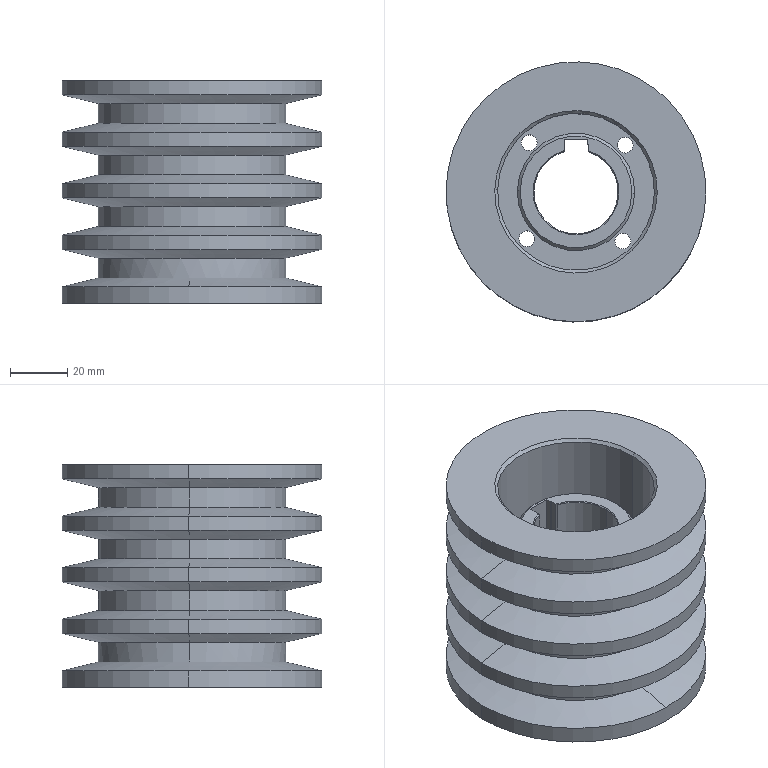Component | SolidWorks | DrivePulley-1 | 1 solid | 80 faces | volume 240587 mm3 | cylinder 37 | cone 30 | plane 13 | commonest cylinder face diameters 90.726 x10 5.517 x8 65.536 x8 41.021 x4 54.753 x4 29.4 x3